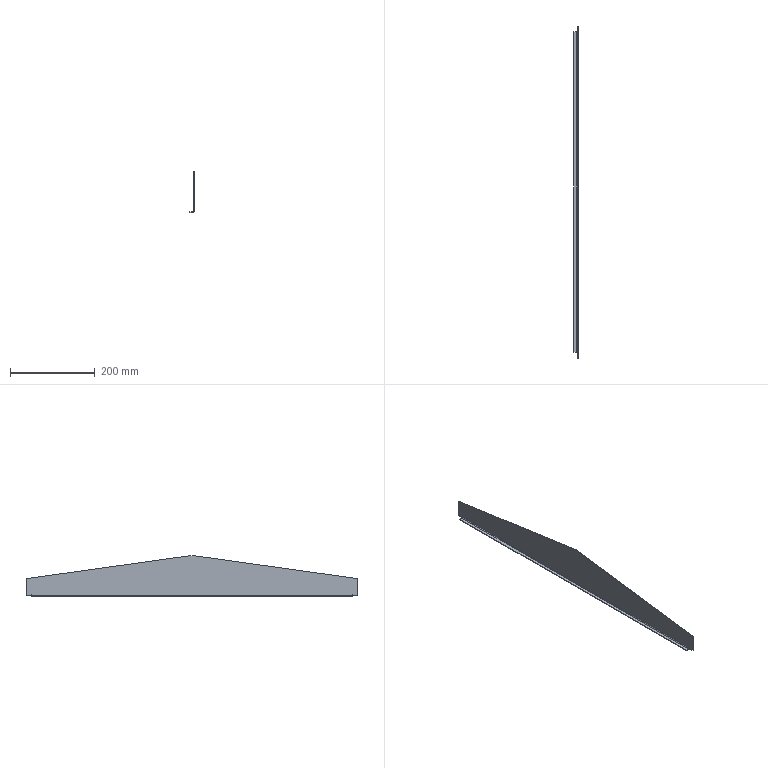Component | SolidWorks | TopCoverAssembly-1_TopCoverEndPlate-1 | 1 solid | 23 faces | box 10 x 784 x 97 mm | volume 90393 mm3 | plane 21 | cylinder 2 | commonest cylinder face diameters 6 x1 3 x1
STEP:
#1=CARTESIAN_POINT('',(25.059,14.945,43.11));
#2=VERTEX_POINT('',#1);
#3=CARTESIAN_POINT('',(25.059,15.427,43.11));
#4=VERTEX_POINT('',#3);
#5=CARTESIAN_POINT('',(25.059,15.427,43.11));
#6=DIRECTION('',(0.,1.,0.));
#7=VECTOR('',#6,39.37);
#8=LINE('',#5,#7);
#9=EDGE_CURVE('',#2,#4,#8,.T.);
#10=ORIENTED_EDGE('',*,*,#9,.F.);
#11=CARTESIAN_POINT('',(25.,14.945,43.11));
#12=VERTEX_POINT('',#11);
#13=CARTESIAN_POINT('',(25.,14.945,43.11));
#14=DIRECTION('',(-1.,0.,0.));
#15=VECTOR('',#14,39.37);
#16=LINE('',#13,#15);
#17=EDGE_CURVE('',#2,#12,#16,.T.);
#18=ORIENTED_EDGE('',*,*,#17,.T.);
#19=CARTESIAN_POINT('',(25.,15.427,43.11));
#20=VERTEX_POINT('',#19);
#21=CARTESIAN_POINT('',(25.,15.427,43.11));
#22=DIRECTION('',(0.,1.,0.));
#23=VECTOR('',#22,39.37);
#24=LINE('',#21,#23);
#25=EDGE_CURVE('',#12,#20,#24,.T.);
#26=ORIENTED_EDGE('',*,*,#25,.T.);
#27=CARTESIAN_POINT('',(25.,15.427,43.11));
#28=DIRECTION('',(1.,-0.,-0.));
#29=VECTOR('',#28,39.37);
#30=LINE('',#27,#29);
#31=EDGE_CURVE('',#20,#4,#30,.T.);
#32=ORIENTED_EDGE('',*,*,#31,.T.);
#33=EDGE_LOOP('',(#10,#18,#26,#32));
#34=FACE_OUTER_BOUND('',#33,.T.);
#35=CARTESIAN_POINT('',(25.,15.427,43.11));
#36=DIRECTION('',(-0.,0.,-1.));
#37=DIRECTION('',(-1.,0.,0.));
#38=AXIS2_PLACEMENT_3D('',#35,#36,#37);
#39=PLANE('',#38);
#40=ADVANCED_FACE('',(#34),#39,.T.);
#41=CARTESIAN_POINT('',(25.,-15.439,43.11));
#42=VERTEX_POINT('',#41);
#43=CARTESIAN_POINT('',(25.,-14.957,43.11));
#44=VERTEX_POINT('',#43);
#45=CARTESIAN_POINT('',(25.,-15.439,43.11));
#46=DIRECTION('',(0.,1.,0.));
#47=VECTOR('',#46,39.37);
#48=LINE('',#45,#47);
#49=EDGE_CURVE('',#42,#44,#48,.T.);
#50=ORIENTED_EDGE('',*,*,#49,.T.);
#51=CARTESIAN_POINT('',(25.059,-14.957,43.11));
#52=VERTEX_POINT('',#51);
#53=CARTESIAN_POINT('',(25.,-14.957,43.11));
#54=DIRECTION('',(1.,-0.,-0.));
#55=VECTOR('',#54,39.37);
#56=LINE('',#53,#55);
#57=EDGE_CURVE('',#44,#52,#56,.T.);
#58=ORIENTED_EDGE('',*,*,#57,.T.);
#59=CARTESIAN_POINT('',(25.059,-15.439,43.11));
#60=VERTEX_POINT('',#59);
#61=CARTESIAN_POINT('',(25.059,-15.439,43.11));
#62=DIRECTION('',(0.,1.,0.));
#63=VECTOR('',#62,39.37);
#64=LINE('',#61,#63);
#65=EDGE_CURVE('',#60,#52,#64,.T.);
#66=ORIENTED_EDGE('',*,*,#65,.F.);
#67=CARTESIAN_POINT('',(25.,-15.439,43.11));
#68=DIRECTION('',(1.,-0.,-0.));
#69=VECTOR('',#68,39.37);
#70=LINE('',#67,#69);
#71=EDGE_CURVE('',#42,#60,#70,.T.);
#72=ORIENTED_EDGE('',*,*,#71,.F.);
#73=EDGE_LOOP('',(#50,#58,#66,#72));
#74=FACE_OUTER_BOUND('',#73,.T.);
#75=CARTESIAN_POINT('',(25.,-15.439,43.11));
#76=DIRECTION('',(-0.,0.,-1.));
#77=DIRECTION('',(-1.,0.,0.));
#78=AXIS2_PLACEMENT_3D('',#75,#76,#77);
#79=PLANE('',#78);
#80=ADVANCED_FACE('',(#74),#79,.T.);
#81=CARTESIAN_POINT('',(25.,-14.957,43.179));
#82=VERTEX_POINT('',#81);
#83=CARTESIAN_POINT('',(25.,-14.957,43.031));
#84=DIRECTION('',(0.,-0.,1.));
#85=VECTOR('',#84,39.37);
#86=LINE('',#83,#85);
#87=EDGE_CURVE('',#44,#82,#86,.T.);
#88=ORIENTED_EDGE('',*,*,#87,.F.);
#89=ORIENTED_EDGE('',*,*,#49,.F.);
#90=CARTESIAN_POINT('',(25.,-15.439,44.697));
#91=VERTEX_POINT('',#90);
#92=CARTESIAN_POINT('',(25.,-15.439,44.697));
#93=DIRECTION('',(-0.,0.,-1.));
#94=VECTOR('',#93,39.37);
#95=LINE('',#92,#94);
#96=EDGE_CURVE('',#91,#42,#95,.T.);
#97=ORIENTED_EDGE('',*,*,#96,.F.);
#98=CARTESIAN_POINT('',(25.,-0.005826,46.85));
#99=VERTEX_POINT('',#98);
#100=CARTESIAN_POINT('',(25.,-0.005826,46.85));
#101=DIRECTION('',(-0.,-0.9904,-0.1382));
#102=VECTOR('',#101,39.37);
#103=LINE('',#100,#102);
#104=EDGE_CURVE('',#99,#91,#103,.T.);
#105=ORIENTED_EDGE('',*,*,#104,.F.);
#106=CARTESIAN_POINT('',(25.,15.427,44.697));
#107=VERTEX_POINT('',#106);
#108=CARTESIAN_POINT('',(25.,15.427,44.697));
#109=DIRECTION('',(-0.,-0.9904,0.1382));
#110=VECTOR('',#109,39.37);
#111=LINE('',#108,#110);
#112=EDGE_CURVE('',#107,#99,#111,.T.);
#113=ORIENTED_EDGE('',*,*,#112,.F.);
#114=CARTESIAN_POINT('',(25.,15.427,43.11));
#115=DIRECTION('',(0.,-0.,1.));
#116=VECTOR('',#115,39.37);
#117=LINE('',#114,#116);
#118=EDGE_CURVE('',#20,#107,#117,.T.);
#119=ORIENTED_EDGE('',*,*,#118,.F.);
#120=ORIENTED_EDGE('',*,*,#25,.F.);
#121=CARTESIAN_POINT('',(25.,14.945,43.179));
#122=VERTEX_POINT('',#121);
#123=CARTESIAN_POINT('',(25.,14.945,43.179));
#124=DIRECTION('',(-0.,0.,-1.));
#125=VECTOR('',#124,39.37);
#126=LINE('',#123,#125);
#127=EDGE_CURVE('',#122,#12,#126,.T.);
#128=ORIENTED_EDGE('',*,*,#127,.F.);
#129=CARTESIAN_POINT('',(25.,14.915,43.179));
#130=VERTEX_POINT('',#129);
#131=CARTESIAN_POINT('',(25.,14.915,43.179));
#132=DIRECTION('',(0.,1.,0.));
#133=VECTOR('',#132,39.37);
#134=LINE('',#131,#133);
#135=EDGE_CURVE('',#130,#122,#134,.T.);
#136=ORIENTED_EDGE('',*,*,#135,.F.);
#137=CARTESIAN_POINT('',(25.,14.915,43.15));
#138=VERTEX_POINT('',#137);
#139=CARTESIAN_POINT('',(25.,14.915,43.15));
#140=DIRECTION('',(0.,-0.,1.));
#141=VECTOR('',#140,39.37);
#142=LINE('',#139,#141);
#143=EDGE_CURVE('',#138,#130,#142,.T.);
#144=ORIENTED_EDGE('',*,*,#143,.F.);
#145=CARTESIAN_POINT('',(25.,-14.927,43.15));
#146=VERTEX_POINT('',#145);
#147=CARTESIAN_POINT('',(25.,-14.927,43.15));
#148=DIRECTION('',(0.,1.,0.));
#149=VECTOR('',#148,39.37);
#150=LINE('',#147,#149);
#151=EDGE_CURVE('',#146,#138,#150,.T.);
#152=ORIENTED_EDGE('',*,*,#151,.F.);
#153=CARTESIAN_POINT('',(25.,-14.927,43.179));
#154=VERTEX_POINT('',#153);
#155=CARTESIAN_POINT('',(25.,-14.927,43.179));
#156=DIRECTION('',(-0.,0.,-1.));
#157=VECTOR('',#156,39.37);
#158=LINE('',#155,#157);
#159=EDGE_CURVE('',#154,#146,#158,.T.);
#160=ORIENTED_EDGE('',*,*,#159,.F.);
#161=CARTESIAN_POINT('',(25.,-14.957,43.179));
#162=DIRECTION('',(0.,1.,0.));
#163=VECTOR('',#162,39.37);
#164=LINE('',#161,#163);
#165=EDGE_CURVE('',#82,#154,#164,.T.);
#166=ORIENTED_EDGE('',*,*,#165,.F.);
#167=EDGE_LOOP('',(#88,#89,#97,#105,#113,#119,#120,#128,#136,#144,#152,#160,#166));
#168=FACE_OUTER_BOUND('',#167,.T.);
#169=CARTESIAN_POINT('',(25.,-15.439,49.004));
#170=DIRECTION('',(1.,-0.,-0.));
#171=DIRECTION('',(-0.,0.,-1.));
#172=AXIS2_PLACEMENT_3D('',#169,#170,#171);
#173=PLANE('',#172);
#174=ADVANCED_FACE('',(#168),#173,.F.);
#175=ORIENTED_EDGE('',*,*,#65,.T.);
#176=CARTESIAN_POINT('',(25.059,-14.957,43.179));
#177=VERTEX_POINT('',#176);
#178=CARTESIAN_POINT('',(25.059,-14.957,49.004));
#179=DIRECTION('',(0.,-0.,1.));
#180=VECTOR('',#179,39.37);
#181=LINE('',#178,#180);
#182=EDGE_CURVE('',#52,#177,#181,.T.);
#183=ORIENTED_EDGE('',*,*,#182,.T.);
#184=CARTESIAN_POINT('',(25.059,-14.927,43.179));
#185=VERTEX_POINT('',#184);
#186=CARTESIAN_POINT('',(25.059,-15.439,43.179));
#187=DIRECTION('',(0.,1.,0.));
#188=VECTOR('',#187,39.37);
#189=LINE('',#186,#188);
#190=EDGE_CURVE('',#177,#185,#189,.T.);
#191=ORIENTED_EDGE('',*,*,#190,.T.);
#192=CARTESIAN_POINT('',(25.059,-14.927,43.15));
#193=VERTEX_POINT('',#192);
#194=CARTESIAN_POINT('',(25.059,-14.927,49.004));
#195=DIRECTION('',(-0.,0.,-1.));
#196=VECTOR('',#195,39.37);
#197=LINE('',#194,#196);
#198=EDGE_CURVE('',#185,#193,#197,.T.);
#199=ORIENTED_EDGE('',*,*,#198,.T.);
#200=CARTESIAN_POINT('',(25.059,14.915,43.15));
#201=VERTEX_POINT('',#200);
#202=CARTESIAN_POINT('',(25.059,-14.927,43.15));
#203=DIRECTION('',(0.,1.,0.));
#204=VECTOR('',#203,39.37);
#205=LINE('',#202,#204);
#206=EDGE_CURVE('',#193,#201,#205,.T.);
#207=ORIENTED_EDGE('',*,*,#206,.T.);
#208=CARTESIAN_POINT('',(25.059,14.915,43.179));
#209=VERTEX_POINT('',#208);
#210=CARTESIAN_POINT('',(25.059,14.915,49.004));
#211=DIRECTION('',(0.,-0.,1.));
#212=VECTOR('',#211,39.37);
#213=LINE('',#210,#212);
#214=EDGE_CURVE('',#201,#209,#213,.T.);
#215=ORIENTED_EDGE('',*,*,#214,.T.);
#216=CARTESIAN_POINT('',(25.059,14.945,43.179));
#217=VERTEX_POINT('',#216);
#218=CARTESIAN_POINT('',(25.059,-15.439,43.179));
#219=DIRECTION('',(0.,1.,0.));
#220=VECTOR('',#219,39.37);
#221=LINE('',#218,#220);
#222=EDGE_CURVE('',#209,#217,#221,.T.);
#223=ORIENTED_EDGE('',*,*,#222,.T.);
#224=CARTESIAN_POINT('',(25.059,14.945,49.004));
#225=DIRECTION('',(-0.,0.,-1.));
#226=VECTOR('',#225,39.37);
#227=LINE('',#224,#226);
#228=EDGE_CURVE('',#217,#2,#227,.T.);
#229=ORIENTED_EDGE('',*,*,#228,.T.);
#230=ORIENTED_EDGE('',*,*,#9,.T.);
#231=CARTESIAN_POINT('',(25.059,15.427,44.697));
#232=VERTEX_POINT('',#231);
#233=CARTESIAN_POINT('',(25.059,15.427,43.11));
#234=DIRECTION('',(0.,-0.,1.));
#235=VECTOR('',#234,39.37);
#236=LINE('',#233,#235);
#237=EDGE_CURVE('',#4,#232,#236,.T.);
#238=ORIENTED_EDGE('',*,*,#237,.T.);
#239=CARTESIAN_POINT('',(25.059,-0.005826,46.85));
#240=VERTEX_POINT('',#239);
#241=CARTESIAN_POINT('',(25.059,15.427,44.697));
#242=DIRECTION('',(-0.,-0.9904,0.1382));
#243=VECTOR('',#242,39.37);
#244=LINE('',#241,#243);
#245=EDGE_CURVE('',#232,#240,#244,.T.);
#246=ORIENTED_EDGE('',*,*,#245,.T.);
#247=CARTESIAN_POINT('',(25.059,-15.439,44.697));
#248=VERTEX_POINT('',#247);
#249=CARTESIAN_POINT('',(25.059,-0.005826,46.85));
#250=DIRECTION('',(-0.,-0.9904,-0.1382));
#251=VECTOR('',#250,39.37);
#252=LINE('',#249,#251);
#253=EDGE_CURVE('',#240,#248,#252,.T.);
#254=ORIENTED_EDGE('',*,*,#253,.T.);
#255=CARTESIAN_POINT('',(25.059,-15.439,44.697));
#256=DIRECTION('',(-0.,0.,-1.));
#257=VECTOR('',#256,39.37);
#258=LINE('',#255,#257);
#259=EDGE_CURVE('',#248,#60,#258,.T.);
#260=ORIENTED_EDGE('',*,*,#259,.T.);
#261=EDGE_LOOP('',(#175,#183,#191,#199,#207,#215,#223,#229,#230,#238,#246,#254,#260));
#262=FACE_OUTER_BOUND('',#261,.T.);
#263=CARTESIAN_POINT('',(25.059,-15.439,49.004));
#264=DIRECTION('',(1.,-0.,-0.));
#265=DIRECTION('',(-0.,0.,-1.));
#266=AXIS2_PLACEMENT_3D('',#263,#264,#265);
#267=PLANE('',#266);
#268=ADVANCED_FACE('',(#262),#267,.T.);
#269=ORIENTED_EDGE('',*,*,#245,.F.);
#270=CARTESIAN_POINT('',(25.,15.427,44.697));
#271=DIRECTION('',(1.,-0.,-0.));
#272=VECTOR('',#271,39.37);
#273=LINE('',#270,#272);
#274=EDGE_CURVE('',#107,#232,#273,.T.);
#275=ORIENTED_EDGE('',*,*,#274,.F.);
#276=ORIENTED_EDGE('',*,*,#112,.T.);
#277=CARTESIAN_POINT('',(25.,-0.005826,46.85));
#278=DIRECTION('',(1.,-0.,-0.));
#279=VECTOR('',#278,39.37);
#280=LINE('',#277,#279);
#281=EDGE_CURVE('',#99,#240,#280,.T.);
#282=ORIENTED_EDGE('',*,*,#281,.T.);
#283=EDGE_LOOP('',(#269,#275,#276,#282));
#284=FACE_OUTER_BOUND('',#283,.T.);
#285=CARTESIAN_POINT('',(25.,15.427,44.697));
#286=DIRECTION('',(0.,0.1382,0.9904));
#287=DIRECTION('',(-0.,-0.9904,0.1382));
#288=AXIS2_PLACEMENT_3D('',#285,#286,#287);
#289=PLANE('',#288);
#290=ADVANCED_FACE('',(#284),#289,.T.);
#291=ORIENTED_EDGE('',*,*,#237,.F.);
#292=ORIENTED_EDGE('',*,*,#31,.F.);
#293=ORIENTED_EDGE('',*,*,#118,.T.);
#294=ORIENTED_EDGE('',*,*,#274,.T.);
#295=EDGE_LOOP('',(#291,#292,#293,#294));
#296=FACE_OUTER_BOUND('',#295,.T.);
#297=CARTESIAN_POINT('',(25.,15.427,43.11));
#298=DIRECTION('',(0.,1.,0.));
#299=DIRECTION('',(1.,-0.,-0.));
#300=AXIS2_PLACEMENT_3D('',#297,#298,#299);
#301=PLANE('',#300);
#302=ADVANCED_FACE('',(#296),#301,.T.);
#303=ORIENTED_EDGE('',*,*,#259,.F.);
#304=CARTESIAN_POINT('',(25.,-15.439,44.697));
#305=DIRECTION('',(1.,-0.,-0.));
#306=VECTOR('',#305,39.37);
#307=LINE('',#304,#306);
#308=EDGE_CURVE('',#91,#248,#307,.T.);
#309=ORIENTED_EDGE('',*,*,#308,.F.);
#310=ORIENTED_EDGE('',*,*,#96,.T.);
#311=ORIENTED_EDGE('',*,*,#71,.T.);
#312=EDGE_LOOP('',(#303,#309,#310,#311));
#313=FACE_OUTER_BOUND('',#312,.T.);
#314=CARTESIAN_POINT('',(25.,-15.439,44.697));
#315=DIRECTION('',(-0.,-1.,-0.));
#316=DIRECTION('',(-1.,0.,0.));
#317=AXIS2_PLACEMENT_3D('',#314,#315,#316);
#318=PLANE('',#317);
#319=ADVANCED_FACE('',(#313),#318,.T.);
#320=ORIENTED_EDGE('',*,*,#253,.F.);
#321=ORIENTED_EDGE('',*,*,#281,.F.);
#322=ORIENTED_EDGE('',*,*,#104,.T.);
#323=ORIENTED_EDGE('',*,*,#308,.T.);
#324=EDGE_LOOP('',(#320,#321,#322,#323));
#325=FACE_OUTER_BOUND('',#324,.T.);
#326=CARTESIAN_POINT('',(25.,-0.005826,46.85));
#327=DIRECTION('',(-0.,-0.1382,0.9904));
#328=DIRECTION('',(-0.,-0.9904,-0.1382));
#329=AXIS2_PLACEMENT_3D('',#326,#327,#328);
#330=PLANE('',#329);
#331=ADVANCED_FACE('',(#325),#330,.T.);
#332=ORIENTED_EDGE('',*,*,#57,.F.);
#333=ORIENTED_EDGE('',*,*,#87,.T.);
#334=CARTESIAN_POINT('',(25.,-14.957,43.179));
#335=DIRECTION('',(1.,-0.,-0.));
#336=VECTOR('',#335,39.37);
#337=LINE('',#334,#336);
#338=EDGE_CURVE('',#82,#177,#337,.T.);
#339=ORIENTED_EDGE('',*,*,#338,.T.);
#340=ORIENTED_EDGE('',*,*,#182,.F.);
#341=EDGE_LOOP('',(#332,#333,#339,#340));
#342=FACE_OUTER_BOUND('',#341,.T.);
#343=CARTESIAN_POINT('',(25.,-14.957,43.031));
#344=DIRECTION('',(0.,1.,0.));
#345=DIRECTION('',(1.,-0.,-0.));
#346=AXIS2_PLACEMENT_3D('',#343,#344,#345);
#347=PLANE('',#346);
#348=ADVANCED_FACE('',(#342),#347,.T.);
#349=ORIENTED_EDGE('',*,*,#190,.F.);
#350=ORIENTED_EDGE('',*,*,#338,.F.);
#351=ORIENTED_EDGE('',*,*,#165,.T.);
#352=CARTESIAN_POINT('',(25.,-14.927,43.179));
#353=DIRECTION('',(1.,-0.,-0.));
#354=VECTOR('',#353,39.37);
#355=LINE('',#352,#354);
#356=EDGE_CURVE('',#154,#185,#355,.T.);
#357=ORIENTED_EDGE('',*,*,#356,.T.);
#358=EDGE_LOOP('',(#349,#350,#351,#357));
#359=FACE_OUTER_BOUND('',#358,.T.);
#360=CARTESIAN_POINT('',(25.,-14.957,43.179));
#361=DIRECTION('',(-0.,0.,-1.));
#362=DIRECTION('',(-1.,0.,0.));
#363=AXIS2_PLACEMENT_3D('',#360,#361,#362);
#364=PLANE('',#363);
#365=ADVANCED_FACE('',(#359),#364,.T.);
#366=ORIENTED_EDGE('',*,*,#198,.F.);
#367=ORIENTED_EDGE('',*,*,#356,.F.);
#368=ORIENTED_EDGE('',*,*,#159,.T.);
#369=CARTESIAN_POINT('',(25.,-14.927,43.15));
#370=DIRECTION('',(1.,-0.,-0.));
#371=VECTOR('',#370,39.37);
#372=LINE('',#369,#371);
#373=EDGE_CURVE('',#146,#193,#372,.T.);
#374=ORIENTED_EDGE('',*,*,#373,.T.);
#375=EDGE_LOOP('',(#366,#367,#368,#374));
#376=FACE_OUTER_BOUND('',#375,.T.);
#377=CARTESIAN_POINT('',(25.,-14.927,43.179));
#378=DIRECTION('',(-0.,-1.,-0.));
#379=DIRECTION('',(-1.,0.,0.));
#380=AXIS2_PLACEMENT_3D('',#377,#378,#379);
#381=PLANE('',#380);
#382=ADVANCED_FACE('',(#376),#381,.T.);
#383=ORIENTED_EDGE('',*,*,#214,.F.);
#384=CARTESIAN_POINT('',(25.,14.915,43.15));
#385=DIRECTION('',(1.,-0.,-0.));
#386=VECTOR('',#385,39.37);
#387=LINE('',#384,#386);
#388=EDGE_CURVE('',#138,#201,#387,.T.);
#389=ORIENTED_EDGE('',*,*,#388,.F.);
#390=ORIENTED_EDGE('',*,*,#143,.T.);
#391=CARTESIAN_POINT('',(25.,14.915,43.179));
#392=DIRECTION('',(1.,-0.,-0.));
#393=VECTOR('',#392,39.37);
#394=LINE('',#391,#393);
#395=EDGE_CURVE('',#130,#209,#394,.T.);
#396=ORIENTED_EDGE('',*,*,#395,.T.);
#397=EDGE_LOOP('',(#383,#389,#390,#396));
#398=FACE_OUTER_BOUND('',#397,.T.);
#399=CARTESIAN_POINT('',(25.,14.915,43.15));
#400=DIRECTION('',(0.,1.,0.));
#401=DIRECTION('',(1.,-0.,-0.));
#402=AXIS2_PLACEMENT_3D('',#399,#400,#401);
#403=PLANE('',#402);
#404=ADVANCED_FACE('',(#398),#403,.T.);
#405=ORIENTED_EDGE('',*,*,#222,.F.);
#406=ORIENTED_EDGE('',*,*,#395,.F.);
#407=ORIENTED_EDGE('',*,*,#135,.T.);
#408=CARTESIAN_POINT('',(25.,14.945,43.179));
#409=DIRECTION('',(1.,-0.,-0.));
#410=VECTOR('',#409,39.37);
#411=LINE('',#408,#410);
#412=EDGE_CURVE('',#122,#217,#411,.T.);
#413=ORIENTED_EDGE('',*,*,#412,.T.);
#414=EDGE_LOOP('',(#405,#406,#407,#413));
#415=FACE_OUTER_BOUND('',#414,.T.);
#416=CARTESIAN_POINT('',(25.,14.915,43.179));
#417=DIRECTION('',(-0.,0.,-1.));
#418=DIRECTION('',(-1.,0.,0.));
#419=AXIS2_PLACEMENT_3D('',#416,#417,#418);
#420=PLANE('',#419);
#421=ADVANCED_FACE('',(#415),#420,.T.);
#422=ORIENTED_EDGE('',*,*,#17,.F.);
#423=ORIENTED_EDGE('',*,*,#228,.F.);
#424=ORIENTED_EDGE('',*,*,#412,.F.);
#425=ORIENTED_EDGE('',*,*,#127,.T.);
#426=EDGE_LOOP('',(#422,#423,#424,#425));
#427=FACE_OUTER_BOUND('',#426,.T.);
#428=CARTESIAN_POINT('',(25.,14.945,43.179));
#429=DIRECTION('',(-0.,-1.,-0.));
#430=DIRECTION('',(-1.,0.,0.));
#431=AXIS2_PLACEMENT_3D('',#428,#429,#430);
#432=PLANE('',#431);
#433=ADVANCED_FACE('',(#427),#432,.T.);
#434=CARTESIAN_POINT('',(24.941,14.915,43.091));
#435=VERTEX_POINT('',#434);
#436=CARTESIAN_POINT('',(24.941,14.915,43.031));
#437=VERTEX_POINT('',#436);
#438=CARTESIAN_POINT('',(24.941,14.915,43.031));
#439=DIRECTION('',(0.,0.,-1.));
#440=VECTOR('',#439,39.37);
#441=LINE('',#438,#440);
#442=EDGE_CURVE('',#435,#437,#441,.T.);
#443=ORIENTED_EDGE('',*,*,#442,.F.);
#444=CARTESIAN_POINT('',(24.941,14.915,43.15));
#445=DIRECTION('',(0.,1.,0.));
#446=DIRECTION('',(-1.,0.,0.));
#447=AXIS2_PLACEMENT_3D('',#444,#445,#446);
#448=CIRCLE('',#447,0.05906);
#449=EDGE_CURVE('',#138,#435,#448,.T.);
#450=ORIENTED_EDGE('',*,*,#449,.F.);
#451=ORIENTED_EDGE('',*,*,#388,.T.);
#452=CARTESIAN_POINT('',(24.941,14.915,43.15));
#453=DIRECTION('',(0.,1.,0.));
#454=DIRECTION('',(-1.,0.,0.));
#455=AXIS2_PLACEMENT_3D('',#452,#453,#454);
#456=CIRCLE('',#455,0.1181);
#457=EDGE_CURVE('',#201,#437,#456,.T.);
#458=ORIENTED_EDGE('',*,*,#457,.T.);
#459=EDGE_LOOP('',(#443,#450,#451,#458));
#460=FACE_OUTER_BOUND('',#459,.T.);
#461=CARTESIAN_POINT('',(24.941,14.915,43.15));
#462=DIRECTION('',(0.,1.,0.));
#463=DIRECTION('',(1.,-0.,-0.));
#464=AXIS2_PLACEMENT_3D('',#461,#462,#463);
#465=PLANE('',#464);
#466=ADVANCED_FACE('',(#460),#465,.T.);
#467=CARTESIAN_POINT('',(24.941,-14.927,43.091));
#468=VERTEX_POINT('',#467);
#469=CARTESIAN_POINT('',(24.941,-14.927,43.15));
#470=DIRECTION('',(-0.,-1.,-0.));
#471=DIRECTION('',(-1.,0.,0.));
#472=AXIS2_PLACEMENT_3D('',#469,#470,#471);
#473=CIRCLE('',#472,0.05906);
#474=EDGE_CURVE('',#468,#146,#473,.T.);
#475=ORIENTED_EDGE('',*,*,#474,.F.);
#476=CARTESIAN_POINT('',(24.941,-14.927,43.031));
#477=VERTEX_POINT('',#476);
#478=CARTESIAN_POINT('',(24.941,-14.927,43.091));
#479=DIRECTION('',(0.,0.,-1.));
#480=VECTOR('',#479,39.37);
#481=LINE('',#478,#480);
#482=EDGE_CURVE('',#468,#477,#481,.T.);
#483=ORIENTED_EDGE('',*,*,#482,.T.);
#484=CARTESIAN_POINT('',(24.941,-14.927,43.15));
#485=DIRECTION('',(-0.,-1.,-0.));
#486=DIRECTION('',(-1.,0.,0.));
#487=AXIS2_PLACEMENT_3D('',#484,#485,#486);
#488=CIRCLE('',#487,0.1181);
#489=EDGE_CURVE('',#477,#193,#488,.T.);
#490=ORIENTED_EDGE('',*,*,#489,.T.);
#491=ORIENTED_EDGE('',*,*,#373,.F.);
#492=EDGE_LOOP('',(#475,#483,#490,#491));
#493=FACE_OUTER_BOUND('',#492,.T.);
#494=CARTESIAN_POINT('',(24.941,-14.927,43.15));
#495=DIRECTION('',(0.,1.,0.));
#496=DIRECTION('',(1.,-0.,-0.));
#497=AXIS2_PLACEMENT_3D('',#494,#495,#496);
#498=PLANE('',#497);
#499=ADVANCED_FACE('',(#493),#498,.F.);
#500=ORIENTED_EDGE('',*,*,#206,.F.);
#501=ORIENTED_EDGE('',*,*,#489,.F.);
#502=CARTESIAN_POINT('',(24.941,14.915,43.031));
#503=DIRECTION('',(0.,1.,0.));
#504=VECTOR('',#503,39.37);
#505=LINE('',#502,#504);
#506=EDGE_CURVE('',#477,#437,#505,.T.);
#507=ORIENTED_EDGE('',*,*,#506,.T.);
#508=ORIENTED_EDGE('',*,*,#457,.F.);
#509=EDGE_LOOP('',(#500,#501,#507,#508));
#510=FACE_OUTER_BOUND('',#509,.T.);
#511=CARTESIAN_POINT('',(24.941,-14.927,43.15));
#512=DIRECTION('',(-0.,-1.,-0.));
#513=DIRECTION('',(0.,0.,-1.));
#514=AXIS2_PLACEMENT_3D('',#511,#512,#513);
#515=CYLINDRICAL_SURFACE('',#514,0.1181);
#516=ADVANCED_FACE('',(#510),#515,.T.);
#517=ORIENTED_EDGE('',*,*,#151,.T.);
#518=ORIENTED_EDGE('',*,*,#449,.T.);
#519=CARTESIAN_POINT('',(24.941,14.915,43.091));
#520=DIRECTION('',(-0.,-1.,-0.));
#521=VECTOR('',#520,39.37);
#522=LINE('',#519,#521);
#523=EDGE_CURVE('',#435,#468,#522,.T.);
#524=ORIENTED_EDGE('',*,*,#523,.T.);
#525=ORIENTED_EDGE('',*,*,#474,.T.);
#526=EDGE_LOOP('',(#517,#518,#524,#525));
#527=FACE_OUTER_BOUND('',#526,.T.);
#528=CARTESIAN_POINT('',(24.941,-14.927,43.15));
#529=DIRECTION('',(-0.,-1.,-0.));
#530=DIRECTION('',(0.,0.,-1.));
#531=AXIS2_PLACEMENT_3D('',#528,#529,#530);
#532=CYLINDRICAL_SURFACE('',#531,0.05906);
#533=ADVANCED_FACE('',(#527),#532,.F.);
#534=ORIENTED_EDGE('',*,*,#482,.F.);
#535=CARTESIAN_POINT('',(24.665,-14.927,43.091));
#536=VERTEX_POINT('',#535);
#537=CARTESIAN_POINT('',(24.665,-14.927,43.091));
#538=DIRECTION('',(-1.,0.,-0.));
#539=VECTOR('',#538,39.37);
#540=LINE('',#537,#539);
#541=EDGE_CURVE('',#468,#536,#540,.T.);
#542=ORIENTED_EDGE('',*,*,#541,.T.);
#543=CARTESIAN_POINT('',(24.665,-14.927,43.031));
#544=VERTEX_POINT('',#543);
#545=CARTESIAN_POINT('',(24.665,-14.927,43.031));
#546=DIRECTION('',(-0.,-0.,1.));
#547=VECTOR('',#546,39.37);
#548=LINE('',#545,#547);
#549=EDGE_CURVE('',#544,#536,#548,.T.);
#550=ORIENTED_EDGE('',*,*,#549,.F.);
#551=CARTESIAN_POINT('',(25.,-14.927,43.031));
#552=DIRECTION('',(-1.,0.,-0.));
#553=VECTOR('',#552,39.37);
#554=LINE('',#551,#553);
#555=EDGE_CURVE('',#477,#544,#554,.T.);
#556=ORIENTED_EDGE('',*,*,#555,.F.);
#557=EDGE_LOOP('',(#534,#542,#550,#556));
#558=FACE_OUTER_BOUND('',#557,.T.);
#559=CARTESIAN_POINT('',(24.665,-14.927,43.031));
#560=DIRECTION('',(0.,1.,0.));
#561=DIRECTION('',(0.,-0.,1.));
#562=AXIS2_PLACEMENT_3D('',#559,#560,#561);
#563=PLANE('',#562);
#564=ADVANCED_FACE('',(#558),#563,.F.);
#565=ORIENTED_EDGE('',*,*,#442,.T.);
#566=CARTESIAN_POINT('',(24.665,14.915,43.031));
#567=VERTEX_POINT('',#566);
#568=CARTESIAN_POINT('',(25.,14.915,43.031));
#569=DIRECTION('',(1.,-0.,0.));
#570=VECTOR('',#569,39.37);
#571=LINE('',#568,#570);
#572=EDGE_CURVE('',#567,#437,#571,.T.);
#573=ORIENTED_EDGE('',*,*,#572,.F.);
#574=CARTESIAN_POINT('',(24.665,14.915,43.091));
#575=VERTEX_POINT('',#574);
#576=CARTESIAN_POINT('',(24.665,14.915,43.031));
#577=DIRECTION('',(-0.,-0.,1.));
#578=VECTOR('',#577,39.37);
#579=LINE('',#576,#578);
#580=EDGE_CURVE('',#567,#575,#579,.T.);
#581=ORIENTED_EDGE('',*,*,#580,.T.);
#582=CARTESIAN_POINT('',(25.,14.915,43.091));
#583=DIRECTION('',(1.,-0.,0.));
#584=VECTOR('',#583,39.37);
#585=LINE('',#582,#584);
#586=EDGE_CURVE('',#575,#435,#585,.T.);
#587=ORIENTED_EDGE('',*,*,#586,.T.);
#588=EDGE_LOOP('',(#565,#573,#581,#587));
#589=FACE_OUTER_BOUND('',#588,.T.);
#590=CARTESIAN_POINT('',(25.,14.915,43.031));
#591=DIRECTION('',(-0.,-1.,-0.));
#592=DIRECTION('',(-0.,0.,-1.));
#593=AXIS2_PLACEMENT_3D('',#590,#591,#592);
#594=PLANE('',#593);
#595=ADVANCED_FACE('',(#589),#594,.F.);
#596=ORIENTED_EDGE('',*,*,#506,.F.);
#597=ORIENTED_EDGE('',*,*,#555,.T.);
#598=CARTESIAN_POINT('',(24.665,-14.927,43.031));
#599=DIRECTION('',(0.,1.,0.));
#600=VECTOR('',#599,39.37);
#601=LINE('',#598,#600);
#602=EDGE_CURVE('',#544,#567,#601,.T.);
#603=ORIENTED_EDGE('',*,*,#602,.T.);
#604=ORIENTED_EDGE('',*,*,#572,.T.);
#605=EDGE_LOOP('',(#596,#597,#603,#604));
#606=FACE_OUTER_BOUND('',#605,.T.);
#607=CARTESIAN_POINT('',(25.,-14.927,43.031));
#608=DIRECTION('',(-0.,-0.,1.));
#609=DIRECTION('',(1.,-0.,0.));
#610=AXIS2_PLACEMENT_3D('',#607,#608,#609);
#611=PLANE('',#610);
#612=ADVANCED_FACE('',(#606),#611,.F.);
#613=ORIENTED_EDGE('',*,*,#541,.F.);
#614=ORIENTED_EDGE('',*,*,#523,.F.);
#615=ORIENTED_EDGE('',*,*,#586,.F.);
#616=CARTESIAN_POINT('',(24.665,14.915,43.091));
#617=DIRECTION('',(0.,1.,0.));
#618=VECTOR('',#617,39.37);
#619=LINE('',#616,#618);
#620=EDGE_CURVE('',#536,#575,#619,.T.);
#621=ORIENTED_EDGE('',*,*,#620,.F.);
#622=EDGE_LOOP('',(#613,#614,#615,#621));
#623=FACE_OUTER_BOUND('',#622,.T.);
#624=CARTESIAN_POINT('',(25.,-14.927,43.091));
#625=DIRECTION('',(-0.,-0.,1.));
#626=DIRECTION('',(1.,-0.,0.));
#627=AXIS2_PLACEMENT_3D('',#624,#625,#626);
#628=PLANE('',#627);
#629=ADVANCED_FACE('',(#623),#628,.T.);
#630=ORIENTED_EDGE('',*,*,#620,.T.);
#631=ORIENTED_EDGE('',*,*,#580,.F.);
#632=ORIENTED_EDGE('',*,*,#602,.F.);
#633=ORIENTED_EDGE('',*,*,#549,.T.);
#634=EDGE_LOOP('',(#630,#631,#632,#633));
#635=FACE_OUTER_BOUND('',#634,.T.);
#636=CARTESIAN_POINT('',(24.665,14.915,43.031));
#637=DIRECTION('',(1.,-0.,0.));
#638=DIRECTION('',(0.,0.,-1.));
#639=AXIS2_PLACEMENT_3D('',#636,#637,#638);
#640=PLANE('',#639);
#641=ADVANCED_FACE('',(#635),#640,.F.);
#642=CLOSED_SHELL('',(#40,#80,#174,#268,#290,#302,#319,#331,#348,#365,#382,#404,#421,#433,#466,#499,#516,#533,#564,#595,#612,#629,#641));
#643=MANIFOLD_SOLID_BREP('',#642);
#644=CARTESIAN_POINT('',(0.,0.,0.));
#645=DIRECTION('',(0.,0.,1.));
#646=DIRECTION('',(1.,0.,0.));
#647=AXIS2_PLACEMENT_3D('',#644,#645,#646);
#648=(LENGTH_UNIT()NAMED_UNIT(*)SI_UNIT($,.METRE.));
#649=LENGTH_MEASURE_WITH_UNIT(LENGTH_MEASURE(0.0254),#648);
#650=DIMENSIONAL_EXPONENTS(1.,0.,0.,0.,0.,0.,0.);
#651=(CONVERSION_BASED_UNIT('',#649)LENGTH_UNIT()NAMED_UNIT(#650));
#652=UNCERTAINTY_MEASURE_WITH_UNIT(LENGTH_MEASURE(0.00001),#651,'','');
#653=(NAMED_UNIT(*)PLANE_ANGLE_UNIT()SI_UNIT($,.RADIAN.));
#654=(NAMED_UNIT(*)SI_UNIT($,.STERADIAN.)SOLID_ANGLE_UNIT());
#655=(GEOMETRIC_REPRESENTATION_CONTEXT(3)GLOBAL_UNCERTAINTY_ASSIGNED_CONTEXT((#652))GLOBAL_UNIT_ASSIGNED_CONTEXT((#651,#653,#654))REPRESENTATION_CONTEXT('',''));
#656=ADVANCED_BREP_SHAPE_REPRESENTATION('',(#643,#647),#655);
#657=COLOUR_RGB('',0.7922,0.8196,0.9333);
#658=FILL_AREA_STYLE_COLOUR('',#657);
#659=FILL_AREA_STYLE('',(#658));
#660=SURFACE_STYLE_FILL_AREA(#659);
#661=SURFACE_SIDE_STYLE('',(#660));
#662=SURFACE_STYLE_USAGE(.BOTH.,#661);
#663=PRESENTATION_STYLE_ASSIGNMENT((#662));
#664=STYLED_ITEM('',(#663),#643);
#665=(LENGTH_UNIT()NAMED_UNIT(*)SI_UNIT($,.METRE.));
#666=LENGTH_MEASURE_WITH_UNIT(LENGTH_MEASURE(0.0254),#665);
#667=DIMENSIONAL_EXPONENTS(1.,0.,0.,0.,0.,0.,0.);
#668=(CONVERSION_BASED_UNIT('',#666)LENGTH_UNIT()NAMED_UNIT(#667));
#669=UNCERTAINTY_MEASURE_WITH_UNIT(LENGTH_MEASURE(0.00001),#668,'','');
#670=(NAMED_UNIT(*)PLANE_ANGLE_UNIT()SI_UNIT($,.RADIAN.));
#671=(NAMED_UNIT(*)SI_UNIT($,.STERADIAN.)SOLID_ANGLE_UNIT());
#672=(GEOMETRIC_REPRESENTATION_CONTEXT(3)GLOBAL_UNCERTAINTY_ASSIGNED_CONTEXT((#669))GLOBAL_UNIT_ASSIGNED_CONTEXT((#668,#670,#671))REPRESENTATION_CONTEXT('',''));
#673=MECHANICAL_DESIGN_GEOMETRIC_PRESENTATION_REPRESENTATION('',(#664),#672);
#674=PRESENTATION_LAYER_ASSIGNMENT('','',(#664));